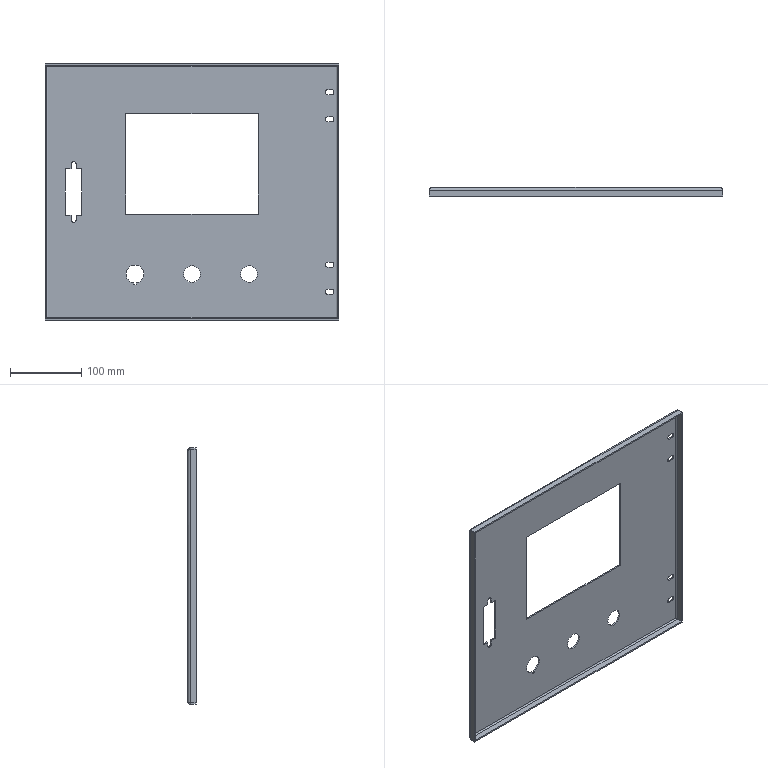Component | SolidWorks | ElectricalCabinetAssembly-1_ControlPanelAssembly-1_ControlPanel-1 | 1 solid | 84 faces | volume 264350 mm3 | plane 47 | cylinder 29 | spline 8 | commonest cylinder face diameters 7 x14 23.3 x4 4 x4 8 x4 25 x3 | material Plain Carbon Steel